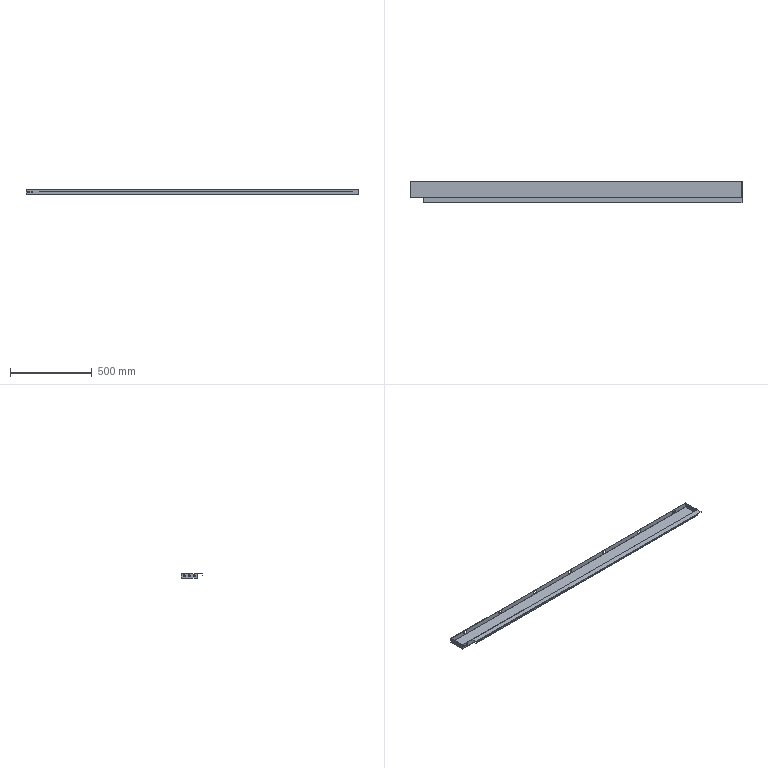Component | SolidWorks | UpperCrossbeam000000-1 | 1 solid | 109 faces | volume 598170 mm3 | plane 64 | cylinder 45 | commonest cylinder face diameters 11 x33 3.4 x6 0.4 x6